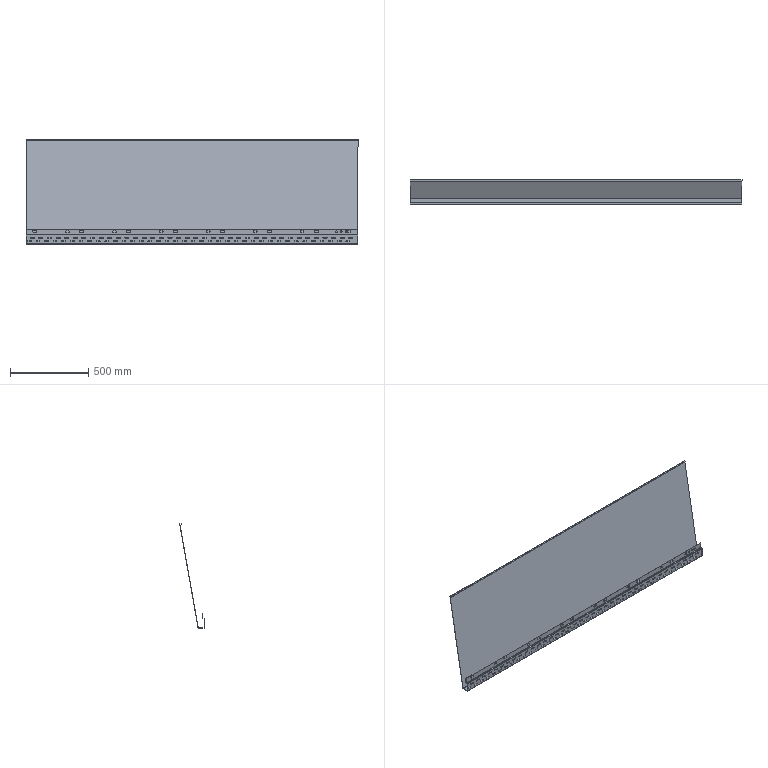Component | SolidWorks | Assembly2-1_TopCoverOne-2 | 1 solid | 412 faces | volume 2607365 mm3 | plane 216 | cylinder 196 | commonest cylinder face diameters 6 x152 11 x34 3.4 x5 0.4 x5